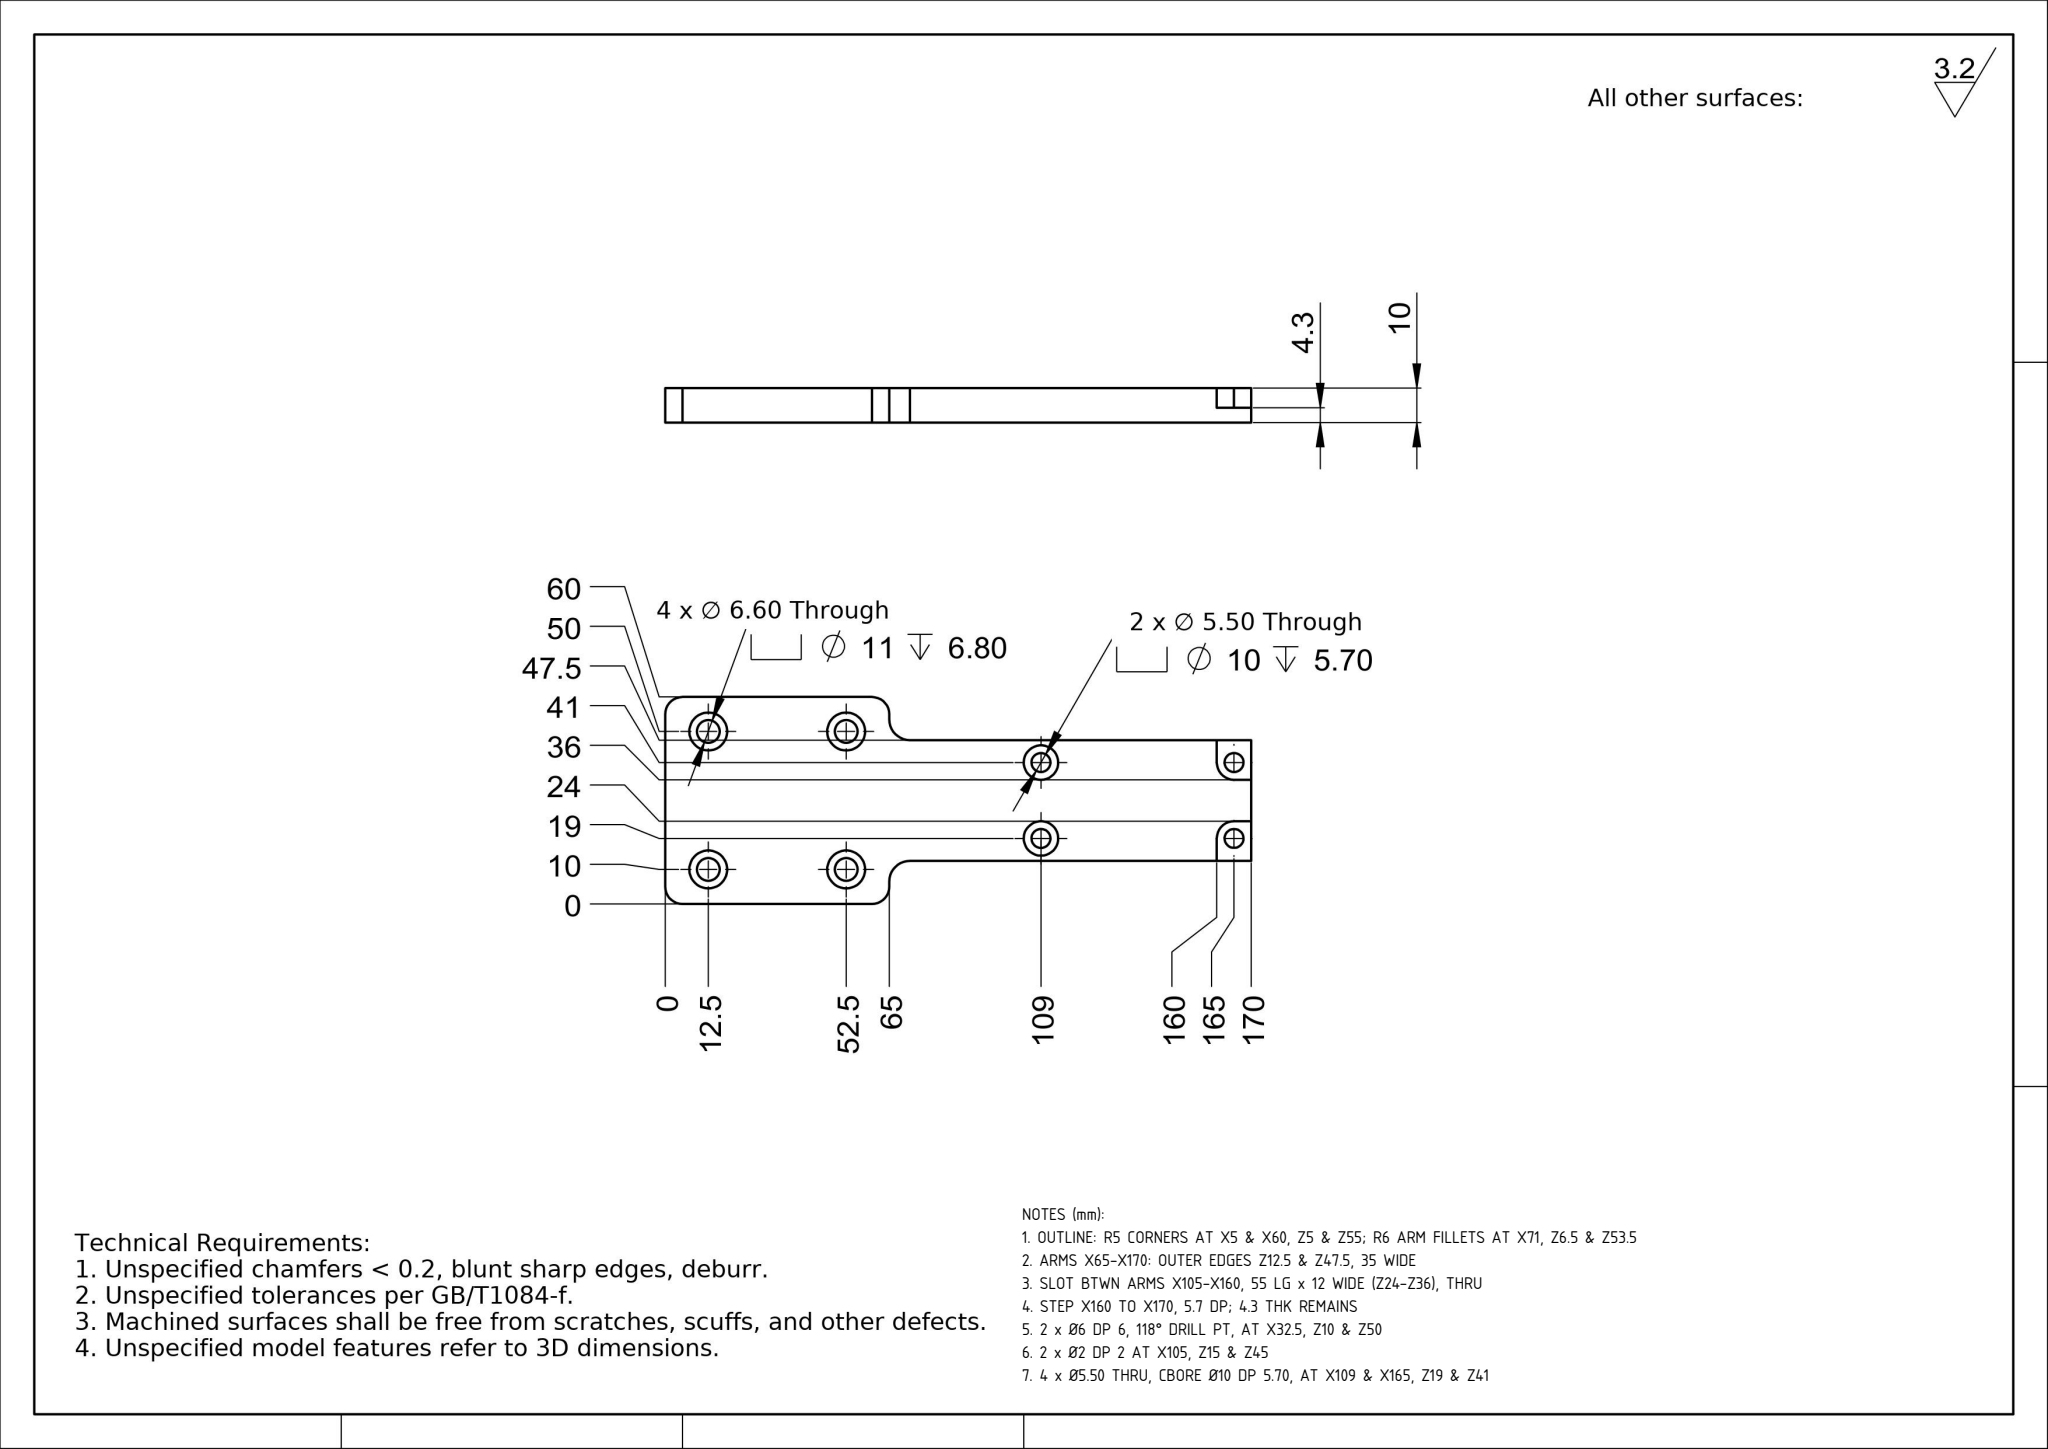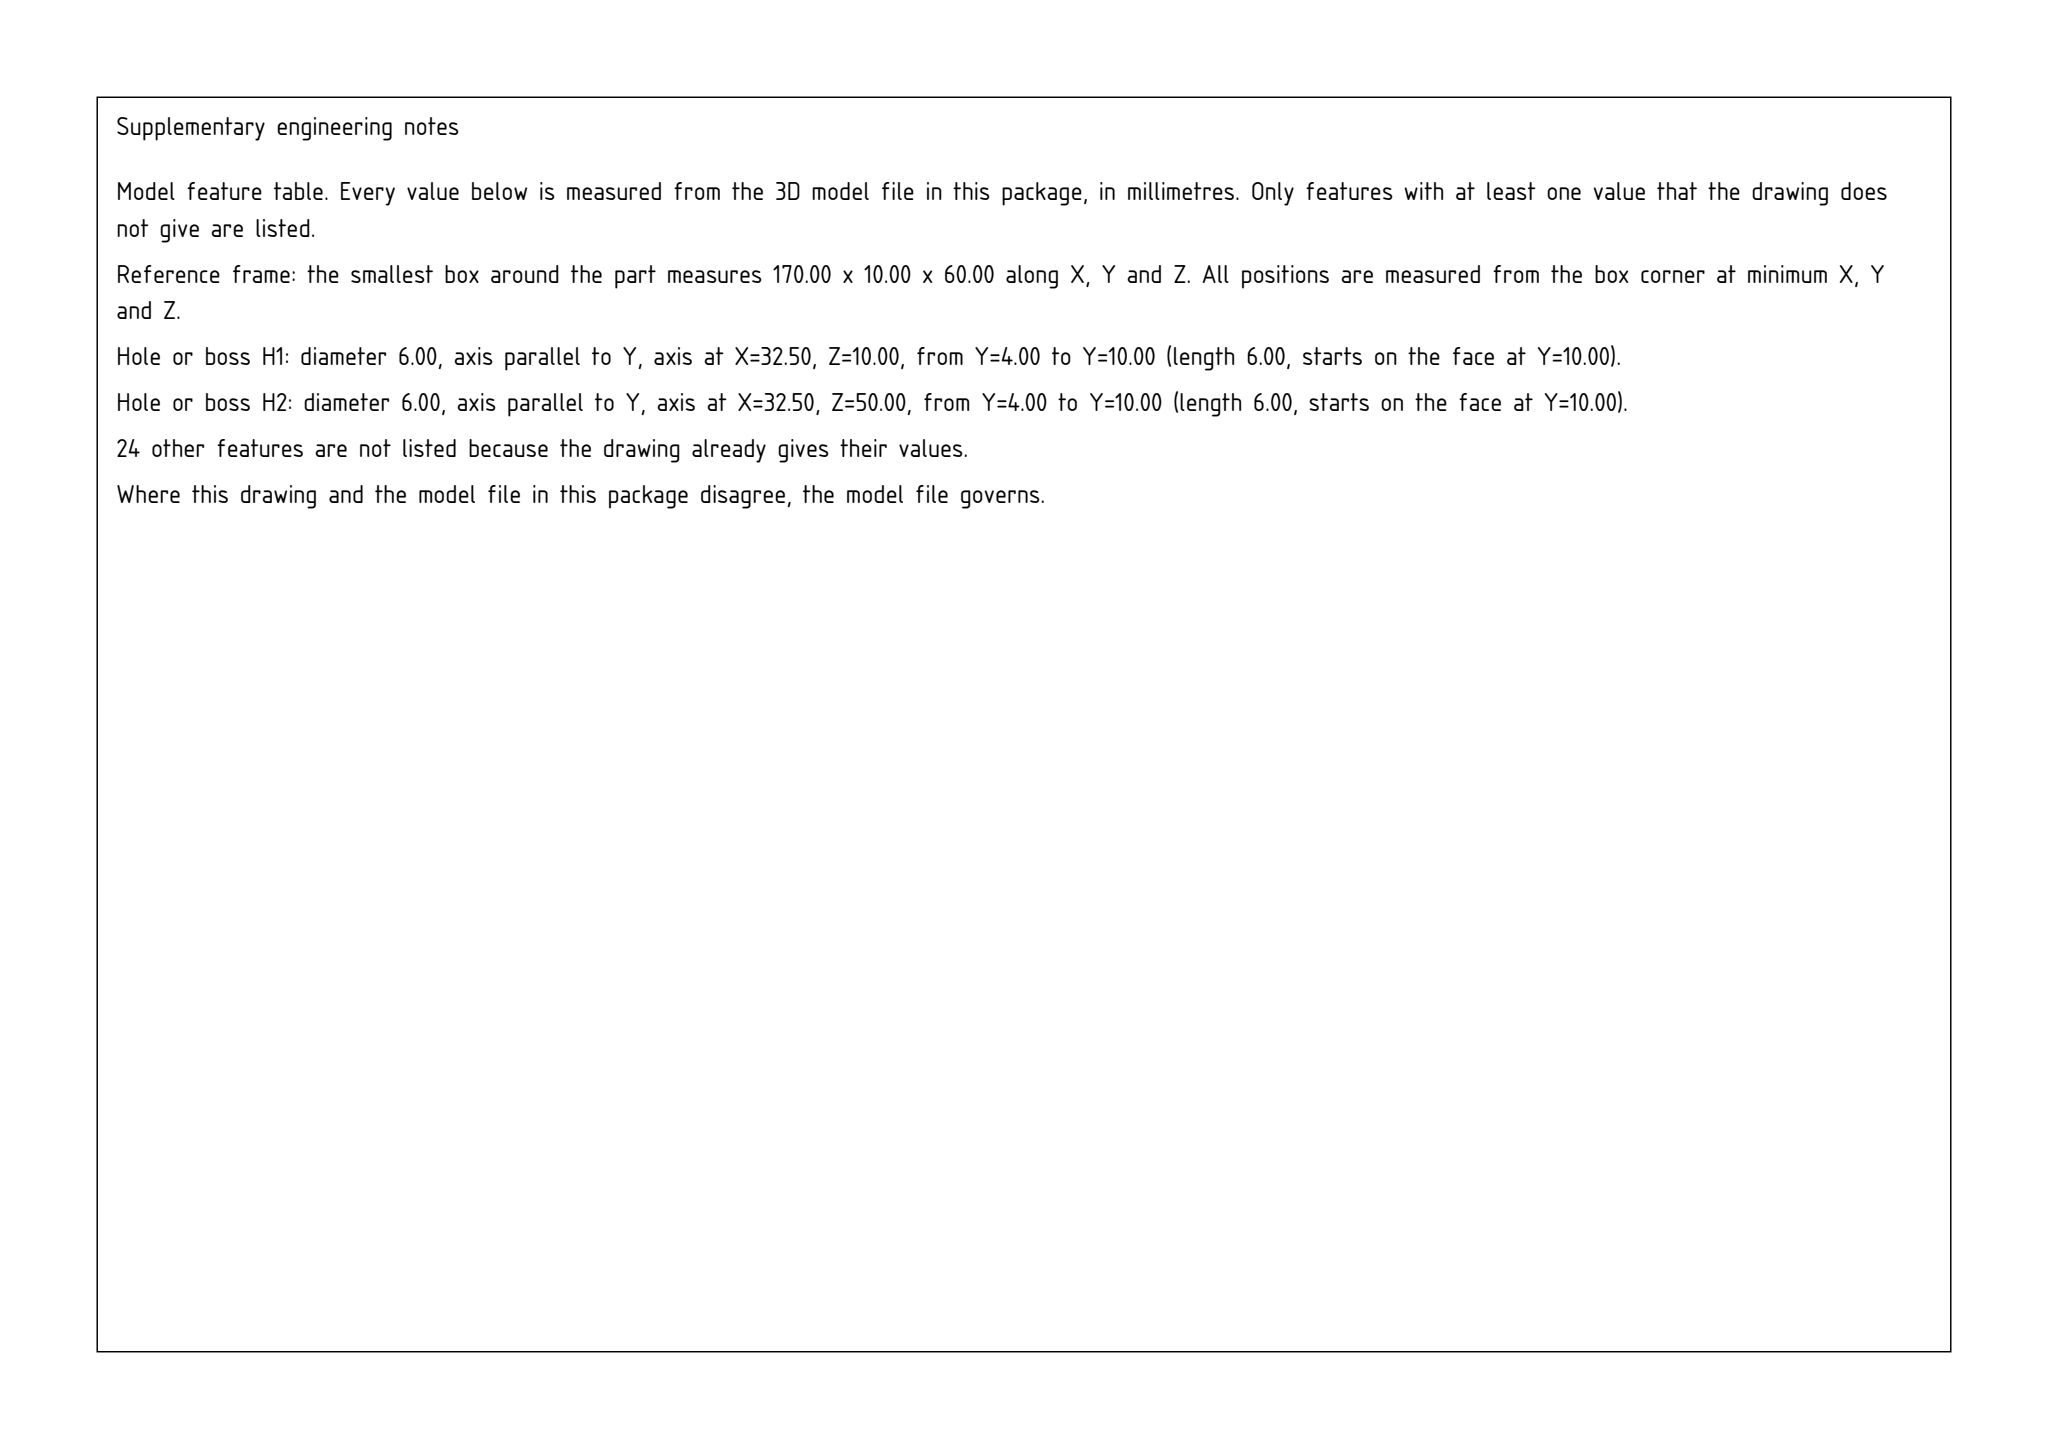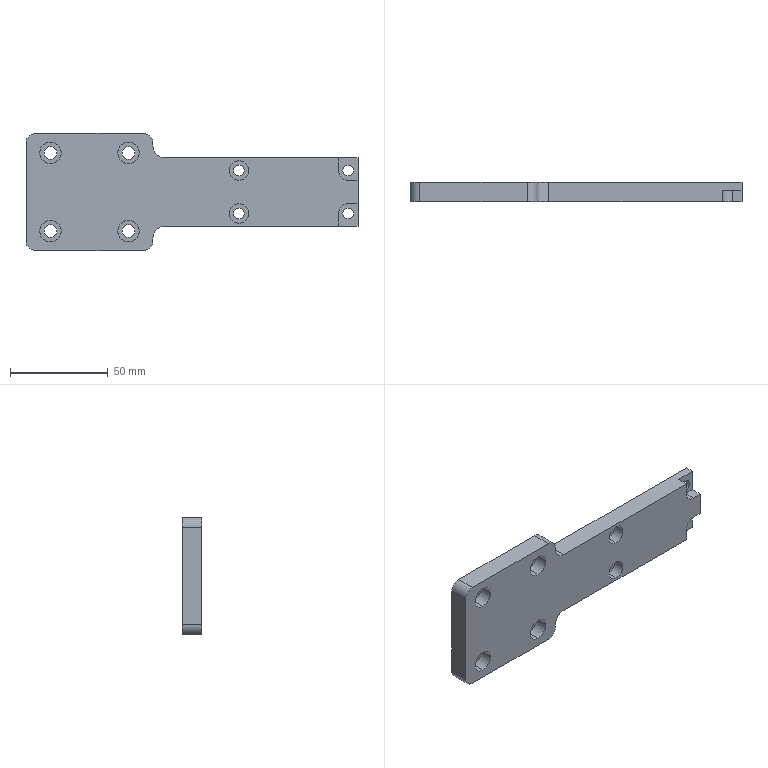Part | SolidWorks | mm | 1 solid | 73 faces | box 170 x 10 x 60 mm | volume 66021 mm3 | cylinder 43 | plane 26 | cone 4 | commonest cylinder face diameters 10 x10 5.5 x8 11 x8 6.6 x8 6 x4 2 x3 12 x2
Drawing notes:
OUTLINE: R5 CORNERS AT X5 & X60, Z5 & Z55; R6 ARM FILLETS AT X71, Z6.5 & Z53.5 | from the solid: Ø10 y-cyl L10 at (5,5),(5,55),(60,5),(60,55)=R5; Ø12 y-cyl L10 at (71,6.5),(71,53.5)=R6
ARMS X65-X170: OUTER EDGES Z12.5 & Z47.5, 35 WIDE | from the solid: z-planes 12.5 & 47.5; x-planes 65 & 170; 47.5-12.5=35
SLOT BTWN ARMS X105-X160, 55 LG x 12 WIDE (Z24-Z36), THRU | from the solid: x-planes 105 & 160 bound opening; z-planes 24/36 = 12 wide; y 0-10 thru
STEP X160 TO X170, 5.7 DP; 4.3 THK REMAINS | from the solid: x-planes 160 (2) & 170; y-planes at 5.7 (4); 10-5.7=4.3
2 x Ø6 DP 6, 118° DRILL PT, AT X32.5, Z10 & Z50 | from the solid: Ø6 y-cyl L6 at (32.5,10) & (32.5,50); cone 118° ref dia 6.0
2 x Ø2 DP 2 AT X105, Z15 & Z45 | from the solid: Ø2 y-cyl L2 at (105,15) & (105,45)
4 x Ø5.50 THRU, CBORE Ø10 DP 5.70, AT X109 & X165, Z19 & Z41 | from the solid: Ø5.5 at (109,19),(109,41),(165,19),(165,41); Ø10 L5.7 at same positions